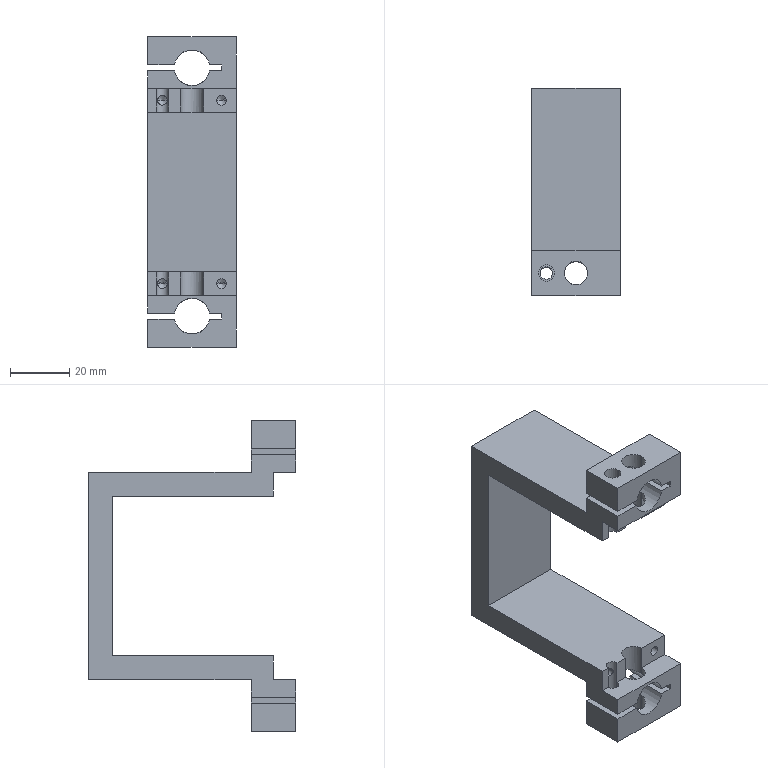Component | SolidWorks | JL001-05-02-1_JL001-05-01-003-1 | 1 solid | 70 faces | box 30 x 70 x 105 mm | volume 52455 mm3 | plane 34 | cylinder 28 | cone 8 | commonest cylinder face diameters 3.3 x8 8 x8 5.5 x4 4.2 x4 12 x4
build123d program:
from build123d import *

# Parameters (mm, degrees)
SKETCH1_W                      = 105
SKETCH1_H                      = 70
BOSS_EXTRUDE1_DEPTH            = 15
SIZE_MM_DOWEL_PIN_HOLE1_D      = 12
SKETCH4_W                      = 2
SKETCH4_H                      = 32
CUT_EXTRUDE1_DEPTH             = 89.776
SKETCH5_W                      = 17.5
SKETCH5_H                      = 55
SKETCH5_W_2                    = 54
SKETCH5_H_2                    = 124
CUT_EXTRUDE2_DEPTH             = 70.866
SIZE_MM_DOWEL_PIN_HOLE2_D      = 8
F_5_5_5_5_DIAMETER_HOLE1_D     = 5.5
F_5_5_5_5_DIAMETER_HOLE1_DEPTH = 11
F_5_5_5_5_DIAMETER_HOLE1_TIP   = 1.652
M5_TAPPED_HOLE1_D              = 4.2
F_5_5_5_5_DIAMETER_HOLE2_D     = 5.5
F_5_5_5_5_DIAMETER_HOLE2_DEPTH = 11
F_5_5_5_5_DIAMETER_HOLE2_TIP   = 1.652
SKETCH14_W                     = 70
SKETCH14_H                     = 30
CUT_EXTRUDE3_DEPTH             = 7.5
M4_TAPPED_HOLE1_D              = 3.3
M4_TAPPED_HOLE1_DEPTH          = 10.1
M4_TAPPED_HOLE1_TIP            = 0.9914


with BuildPart() as part:
    # Sketch1 → Boss-Extrude1 (new, symmetric)
    with BuildSketch(Plane.XY):
        Rectangle(SKETCH1_W, SKETCH1_H)
    extrude(amount=BOSS_EXTRUDE1_DEPTH, both=True)

    # Size mm Dowel Pin Hole1 (through all)
    with Locations(Plane(origin=(0, 35, 0), x_dir=(1, 0, 0), z_dir=(0, 1, 0))):
        with Locations((-42, 0), (42, 0)):
            Hole(SIZE_MM_DOWEL_PIN_HOLE1_D / 2)

    # Sketch4 → Cut-Extrude1 (cut, through all)
    with BuildSketch(Plane(origin=(0, 35, 0), x_dir=(1, 0, 0), z_dir=(0, 1, 0))):
        with Locations((-42, -6)):
            Rectangle(SKETCH4_W, SKETCH4_H)
        with Locations((42, -6)):
            Rectangle(SKETCH4_W, SKETCH4_H)
    extrude(amount=-CUT_EXTRUDE1_DEPTH, mode=Mode.SUBTRACT)

    # Sketch5 → Cut-Extrude2 (cut, through all)
    with BuildSketch(Plane.XY.offset(15)):
        with Locations((-43.75, -7.5)):
            Rectangle(SKETCH5_W, SKETCH5_H)
        with Locations((43.75, -7.5)):
            Rectangle(SKETCH5_W, SKETCH5_H)
        with Locations((0, 35)):
            Rectangle(SKETCH5_W_2, SKETCH5_H_2)
    extrude(amount=-CUT_EXTRUDE2_DEPTH, mode=Mode.SUBTRACT)

    # Size mm Dowel Pin Hole2 (through all)
    with Locations(Plane.ZY.offset(52.5)):
        with Locations((0, 27.5)):
            Hole(SIZE_MM_DOWEL_PIN_HOLE2_D / 2)

    # 5.5 _5.5_ Diameter Hole1
    with Locations(Plane(origin=(52.5, 0, 0), x_dir=(0, 0, -1), z_dir=(1, 0, 0))):
        with Locations((-10, 27.5)):
            Hole(F_5_5_5_5_DIAMETER_HOLE1_D / 2, depth=F_5_5_5_5_DIAMETER_HOLE1_DEPTH)
            with Locations((0, 0, -(F_5_5_5_5_DIAMETER_HOLE1_DEPTH + F_5_5_5_5_DIAMETER_HOLE1_TIP / 2))):  # 118° drill point
                Cone(0, F_5_5_5_5_DIAMETER_HOLE1_D / 2, F_5_5_5_5_DIAMETER_HOLE1_TIP, mode=Mode.SUBTRACT)

    # M5 Tapped Hole1 (through all)
    with Locations(Plane(origin=(41, 0, 0), x_dir=(0, 0, -1), z_dir=(1, 0, 0))):
        with Locations((-10, 27.5)):
            Hole(M5_TAPPED_HOLE1_D / 2)

    # 5.5 _5.5_ Diameter Hole2
    with Locations(Plane.ZY.offset(52.5)):
        with Locations((10, 27.5)):
            Hole(F_5_5_5_5_DIAMETER_HOLE2_D / 2, depth=F_5_5_5_5_DIAMETER_HOLE2_DEPTH)
            with Locations((0, 0, -(F_5_5_5_5_DIAMETER_HOLE2_DEPTH + F_5_5_5_5_DIAMETER_HOLE2_TIP / 2))):  # 118° drill point
                Cone(0, F_5_5_5_5_DIAMETER_HOLE2_D / 2, F_5_5_5_5_DIAMETER_HOLE2_TIP, mode=Mode.SUBTRACT)

    # Sketch14 → Cut-Extrude3 (cut)
    with BuildSketch(Plane(origin=(0, 35, 0), x_dir=(1, 0, 0), z_dir=(0, 1, 0))):
        Rectangle(SKETCH14_W, SKETCH14_H)
    extrude(amount=-CUT_EXTRUDE3_DEPTH, mode=Mode.SUBTRACT)

    # M4 Tapped Hole1
    with Locations(Plane(origin=(0, 27.5, 0), x_dir=(1, 0, 0), z_dir=(0, 1, 0))):
        with Locations((-31, 10), (-31, -10), (31, 10), (31, -10)):
            Hole(M4_TAPPED_HOLE1_D / 2, depth=M4_TAPPED_HOLE1_DEPTH)
            with Locations((0, 0, -(M4_TAPPED_HOLE1_DEPTH + M4_TAPPED_HOLE1_TIP / 2))):  # 118° drill point
                Cone(0, M4_TAPPED_HOLE1_D / 2, M4_TAPPED_HOLE1_TIP, mode=Mode.SUBTRACT)


solid = part.part

# Placed as in the assembly
solid = solid.moved(Location((0, 1075, 63), (180, -90, 0)))